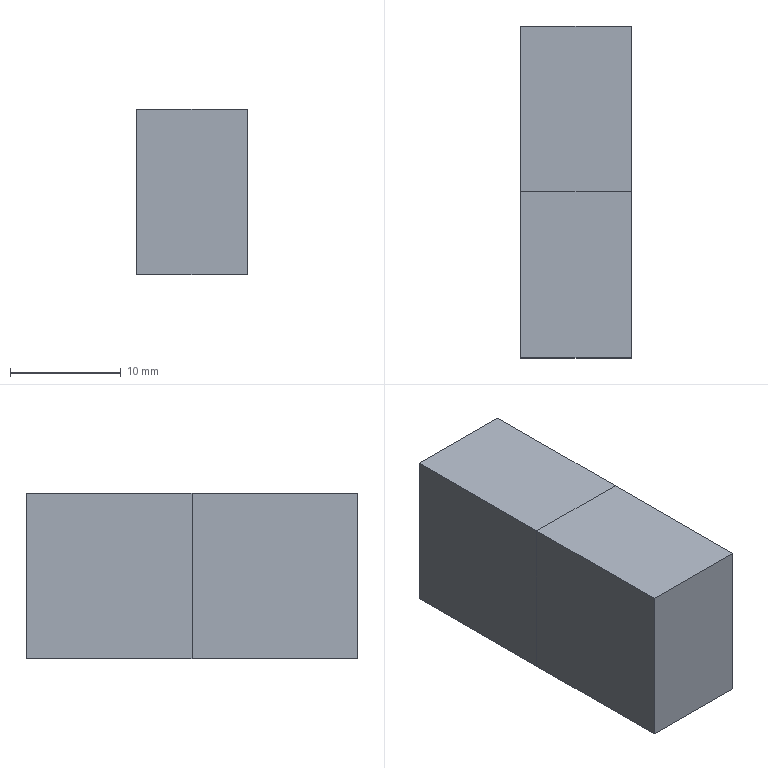Component | NX | 11_OBJECT_4 | 2 solids | 12 faces | box 10 x 30 x 15 mm | volume 4500 mm3 | plane 12
STEP:
#1=CARTESIAN_POINT('',(0.,0.,0.));
#2=DIRECTION('',(0.,0.,1.));
#3=DIRECTION('',(1.,0.,0.));
#4=AXIS2_PLACEMENT_3D('',#1,#2,#3);
#5=CARTESIAN_POINT('',(2050.,34.5,562.5));
#6=VERTEX_POINT('',#5);
#7=CARTESIAN_POINT('',(2050.,49.5,562.5));
#8=VERTEX_POINT('',#7);
#9=CARTESIAN_POINT('',(2050.,34.5,562.5));
#10=DIRECTION('',(0.,1.,0.));
#11=VECTOR('',#10,1.);
#12=LINE('',#9,#11);
#13=CARTESIAN_POINT('',(2060.,34.5,562.5));
#14=DIRECTION('',(0.,0.,1.));
#15=DIRECTION('',(0.,1.,0.));
#16=AXIS2_PLACEMENT_3D('',#13,#14,#15);
#17=PLANE('',#16);
#18=CARTESIAN_POINT('',(0.,10.));
#19=DIRECTION('',(1.,0.));
#20=VECTOR('',#19,1.);
#21=LINE('',#18,#20);
#22=(GEOMETRIC_REPRESENTATION_CONTEXT(2)PARAMETRIC_REPRESENTATION_CONTEXT()REPRESENTATION_CONTEXT('',''));
#23=DEFINITIONAL_REPRESENTATION('',(#21),#22);
#24=PCURVE('',#17,#23);
#25=CARTESIAN_POINT('',(2050.,34.5,562.5));
#26=DIRECTION('',(1.,0.,0.));
#27=DIRECTION('',(0.,1.,0.));
#28=AXIS2_PLACEMENT_3D('',#25,#26,#27);
#29=PLANE('',#28);
#30=CARTESIAN_POINT('',(0.,0.));
#31=DIRECTION('',(1.,0.));
#32=VECTOR('',#31,1.);
#33=LINE('',#30,#32);
#34=(GEOMETRIC_REPRESENTATION_CONTEXT(2)PARAMETRIC_REPRESENTATION_CONTEXT()REPRESENTATION_CONTEXT('',''));
#35=DEFINITIONAL_REPRESENTATION('',(#33),#34);
#36=PCURVE('',#29,#35);
#37=SURFACE_CURVE('',#12,(#24,#36),.PCURVE_S1.);
#38=EDGE_CURVE('',#6,#8,#37,.T.);
#39=ORIENTED_EDGE('',*,*,#38,.T.);
#40=CARTESIAN_POINT('',(2060.,49.5,562.5));
#41=VERTEX_POINT('',#40);
#42=CARTESIAN_POINT('',(2060.,49.5,562.5));
#43=DIRECTION('',(-1.,0.,0.));
#44=VECTOR('',#43,1.);
#45=LINE('',#42,#44);
#46=CARTESIAN_POINT('',(15.,0.));
#47=DIRECTION('',(0.,1.));
#48=VECTOR('',#47,1.);
#49=LINE('',#46,#48);
#50=(GEOMETRIC_REPRESENTATION_CONTEXT(2)PARAMETRIC_REPRESENTATION_CONTEXT()REPRESENTATION_CONTEXT('',''));
#51=DEFINITIONAL_REPRESENTATION('',(#49),#50);
#52=PCURVE('',#17,#51);
#53=CARTESIAN_POINT('',(2060.,49.5,562.5));
#54=DIRECTION('',(0.,-1.,0.));
#55=DIRECTION('',(0.,0.,1.));
#56=AXIS2_PLACEMENT_3D('',#53,#54,#55);
#57=PLANE('',#56);
#58=CARTESIAN_POINT('',(0.,0.));
#59=DIRECTION('',(0.,1.));
#60=VECTOR('',#59,1.);
#61=LINE('',#58,#60);
#62=(GEOMETRIC_REPRESENTATION_CONTEXT(2)PARAMETRIC_REPRESENTATION_CONTEXT()REPRESENTATION_CONTEXT('',''));
#63=DEFINITIONAL_REPRESENTATION('',(#61),#62);
#64=PCURVE('',#57,#63);
#65=SURFACE_CURVE('',#45,(#52,#64),.PCURVE_S1.);
#66=EDGE_CURVE('',#41,#8,#65,.T.);
#67=ORIENTED_EDGE('',*,*,#66,.F.);
#68=CARTESIAN_POINT('',(2060.,34.5,562.5));
#69=VERTEX_POINT('',#68);
#70=CARTESIAN_POINT('',(2060.,34.5,562.5));
#71=DIRECTION('',(0.,1.,0.));
#72=VECTOR('',#71,1.);
#73=LINE('',#70,#72);
#74=CARTESIAN_POINT('',(0.,0.));
#75=DIRECTION('',(1.,0.));
#76=VECTOR('',#75,1.);
#77=LINE('',#74,#76);
#78=(GEOMETRIC_REPRESENTATION_CONTEXT(2)PARAMETRIC_REPRESENTATION_CONTEXT()REPRESENTATION_CONTEXT('',''));
#79=DEFINITIONAL_REPRESENTATION('',(#77),#78);
#80=PCURVE('',#17,#79);
#81=CARTESIAN_POINT('',(2060.,34.5,562.5));
#82=DIRECTION('',(1.,0.,0.));
#83=DIRECTION('',(0.,1.,0.));
#84=AXIS2_PLACEMENT_3D('',#81,#82,#83);
#85=PLANE('',#84);
#86=CARTESIAN_POINT('',(0.,0.));
#87=DIRECTION('',(1.,0.));
#88=VECTOR('',#87,1.);
#89=LINE('',#86,#88);
#90=(GEOMETRIC_REPRESENTATION_CONTEXT(2)PARAMETRIC_REPRESENTATION_CONTEXT()REPRESENTATION_CONTEXT('',''));
#91=DEFINITIONAL_REPRESENTATION('',(#89),#90);
#92=PCURVE('',#85,#91);
#93=SURFACE_CURVE('',#73,(#80,#92),.PCURVE_S1.);
#94=EDGE_CURVE('',#69,#41,#93,.T.);
#95=ORIENTED_EDGE('',*,*,#94,.F.);
#96=CARTESIAN_POINT('',(2060.,34.5,562.5));
#97=DIRECTION('',(-1.,0.,0.));
#98=VECTOR('',#97,1.);
#99=LINE('',#96,#98);
#100=CARTESIAN_POINT('',(0.,0.));
#101=DIRECTION('',(0.,1.));
#102=VECTOR('',#101,1.);
#103=LINE('',#100,#102);
#104=(GEOMETRIC_REPRESENTATION_CONTEXT(2)PARAMETRIC_REPRESENTATION_CONTEXT()REPRESENTATION_CONTEXT('',''));
#105=DEFINITIONAL_REPRESENTATION('',(#103),#104);
#106=PCURVE('',#17,#105);
#107=CARTESIAN_POINT('',(2060.,34.5,577.5));
#108=DIRECTION('',(0.,1.,0.));
#109=DIRECTION('',(0.,0.,-1.));
#110=AXIS2_PLACEMENT_3D('',#107,#108,#109);
#111=PLANE('',#110);
#112=CARTESIAN_POINT('',(15.,0.));
#113=DIRECTION('',(0.,1.));
#114=VECTOR('',#113,1.);
#115=LINE('',#112,#114);
#116=(GEOMETRIC_REPRESENTATION_CONTEXT(2)PARAMETRIC_REPRESENTATION_CONTEXT()REPRESENTATION_CONTEXT('',''));
#117=DEFINITIONAL_REPRESENTATION('',(#115),#116);
#118=PCURVE('',#111,#117);
#119=SURFACE_CURVE('',#99,(#106,#118),.PCURVE_S1.);
#120=EDGE_CURVE('',#69,#6,#119,.T.);
#121=ORIENTED_EDGE('',*,*,#120,.T.);
#122=EDGE_LOOP('',(#39,#67,#95,#121));
#123=FACE_BOUND('',#122,.T.);
#124=ADVANCED_FACE('',(#123),#17,.F.);
#125=CARTESIAN_POINT('',(2050.,49.5,577.5));
#126=VERTEX_POINT('',#125);
#127=CARTESIAN_POINT('',(2050.,49.5,562.5));
#128=DIRECTION('',(0.,0.,1.));
#129=VECTOR('',#128,1.);
#130=LINE('',#127,#129);
#131=CARTESIAN_POINT('',(0.,10.));
#132=DIRECTION('',(1.,0.));
#133=VECTOR('',#132,1.);
#134=LINE('',#131,#133);
#135=(GEOMETRIC_REPRESENTATION_CONTEXT(2)PARAMETRIC_REPRESENTATION_CONTEXT()REPRESENTATION_CONTEXT('',''));
#136=DEFINITIONAL_REPRESENTATION('',(#134),#135);
#137=PCURVE('',#57,#136);
#138=CARTESIAN_POINT('',(15.,0.));
#139=DIRECTION('',(0.,1.));
#140=VECTOR('',#139,1.);
#141=LINE('',#138,#140);
#142=(GEOMETRIC_REPRESENTATION_CONTEXT(2)PARAMETRIC_REPRESENTATION_CONTEXT()REPRESENTATION_CONTEXT('',''));
#143=DEFINITIONAL_REPRESENTATION('',(#141),#142);
#144=PCURVE('',#29,#143);
#145=SURFACE_CURVE('',#130,(#137,#144),.PCURVE_S1.);
#146=EDGE_CURVE('',#8,#126,#145,.T.);
#147=ORIENTED_EDGE('',*,*,#146,.T.);
#148=CARTESIAN_POINT('',(2060.,49.5,577.5));
#149=VERTEX_POINT('',#148);
#150=CARTESIAN_POINT('',(2060.,49.5,577.5));
#151=DIRECTION('',(-1.,0.,0.));
#152=VECTOR('',#151,1.);
#153=LINE('',#150,#152);
#154=CARTESIAN_POINT('',(15.,0.));
#155=DIRECTION('',(0.,1.));
#156=VECTOR('',#155,1.);
#157=LINE('',#154,#156);
#158=(GEOMETRIC_REPRESENTATION_CONTEXT(2)PARAMETRIC_REPRESENTATION_CONTEXT()REPRESENTATION_CONTEXT('',''));
#159=DEFINITIONAL_REPRESENTATION('',(#157),#158);
#160=PCURVE('',#57,#159);
#161=CARTESIAN_POINT('',(2060.,49.5,577.5));
#162=DIRECTION('',(0.,0.,-1.));
#163=DIRECTION('',(0.,-1.,0.));
#164=AXIS2_PLACEMENT_3D('',#161,#162,#163);
#165=PLANE('',#164);
#166=CARTESIAN_POINT('',(0.,0.));
#167=DIRECTION('',(0.,1.));
#168=VECTOR('',#167,1.);
#169=LINE('',#166,#168);
#170=(GEOMETRIC_REPRESENTATION_CONTEXT(2)PARAMETRIC_REPRESENTATION_CONTEXT()REPRESENTATION_CONTEXT('',''));
#171=DEFINITIONAL_REPRESENTATION('',(#169),#170);
#172=PCURVE('',#165,#171);
#173=SURFACE_CURVE('',#153,(#160,#172),.PCURVE_S1.);
#174=EDGE_CURVE('',#149,#126,#173,.T.);
#175=ORIENTED_EDGE('',*,*,#174,.F.);
#176=CARTESIAN_POINT('',(2060.,49.5,562.5));
#177=DIRECTION('',(0.,0.,1.));
#178=VECTOR('',#177,1.);
#179=LINE('',#176,#178);
#180=CARTESIAN_POINT('',(0.,0.));
#181=DIRECTION('',(1.,0.));
#182=VECTOR('',#181,1.);
#183=LINE('',#180,#182);
#184=(GEOMETRIC_REPRESENTATION_CONTEXT(2)PARAMETRIC_REPRESENTATION_CONTEXT()REPRESENTATION_CONTEXT('',''));
#185=DEFINITIONAL_REPRESENTATION('',(#183),#184);
#186=PCURVE('',#57,#185);
#187=CARTESIAN_POINT('',(15.,0.));
#188=DIRECTION('',(0.,1.));
#189=VECTOR('',#188,1.);
#190=LINE('',#187,#189);
#191=(GEOMETRIC_REPRESENTATION_CONTEXT(2)PARAMETRIC_REPRESENTATION_CONTEXT()REPRESENTATION_CONTEXT('',''));
#192=DEFINITIONAL_REPRESENTATION('',(#190),#191);
#193=PCURVE('',#85,#192);
#194=SURFACE_CURVE('',#179,(#186,#193),.PCURVE_S1.);
#195=EDGE_CURVE('',#41,#149,#194,.T.);
#196=ORIENTED_EDGE('',*,*,#195,.F.);
#197=ORIENTED_EDGE('',*,*,#66,.T.);
#198=EDGE_LOOP('',(#147,#175,#196,#197));
#199=FACE_BOUND('',#198,.T.);
#200=ADVANCED_FACE('',(#199),#57,.F.);
#201=CARTESIAN_POINT('',(2050.,34.5,577.5));
#202=VERTEX_POINT('',#201);
#203=CARTESIAN_POINT('',(2050.,49.5,577.5));
#204=DIRECTION('',(0.,-1.,0.));
#205=VECTOR('',#204,1.);
#206=LINE('',#203,#205);
#207=CARTESIAN_POINT('',(0.,10.));
#208=DIRECTION('',(1.,0.));
#209=VECTOR('',#208,1.);
#210=LINE('',#207,#209);
#211=(GEOMETRIC_REPRESENTATION_CONTEXT(2)PARAMETRIC_REPRESENTATION_CONTEXT()REPRESENTATION_CONTEXT('',''));
#212=DEFINITIONAL_REPRESENTATION('',(#210),#211);
#213=PCURVE('',#165,#212);
#214=CARTESIAN_POINT('',(15.,15.));
#215=DIRECTION('',(-1.,0.));
#216=VECTOR('',#215,1.);
#217=LINE('',#214,#216);
#218=(GEOMETRIC_REPRESENTATION_CONTEXT(2)PARAMETRIC_REPRESENTATION_CONTEXT()REPRESENTATION_CONTEXT('',''));
#219=DEFINITIONAL_REPRESENTATION('',(#217),#218);
#220=PCURVE('',#29,#219);
#221=SURFACE_CURVE('',#206,(#213,#220),.PCURVE_S1.);
#222=EDGE_CURVE('',#126,#202,#221,.T.);
#223=ORIENTED_EDGE('',*,*,#222,.T.);
#224=CARTESIAN_POINT('',(2060.,34.5,577.5));
#225=VERTEX_POINT('',#224);
#226=CARTESIAN_POINT('',(2060.,34.5,577.5));
#227=DIRECTION('',(-1.,0.,0.));
#228=VECTOR('',#227,1.);
#229=LINE('',#226,#228);
#230=CARTESIAN_POINT('',(15.,0.));
#231=DIRECTION('',(0.,1.));
#232=VECTOR('',#231,1.);
#233=LINE('',#230,#232);
#234=(GEOMETRIC_REPRESENTATION_CONTEXT(2)PARAMETRIC_REPRESENTATION_CONTEXT()REPRESENTATION_CONTEXT('',''));
#235=DEFINITIONAL_REPRESENTATION('',(#233),#234);
#236=PCURVE('',#165,#235);
#237=CARTESIAN_POINT('',(0.,0.));
#238=DIRECTION('',(0.,1.));
#239=VECTOR('',#238,1.);
#240=LINE('',#237,#239);
#241=(GEOMETRIC_REPRESENTATION_CONTEXT(2)PARAMETRIC_REPRESENTATION_CONTEXT()REPRESENTATION_CONTEXT('',''));
#242=DEFINITIONAL_REPRESENTATION('',(#240),#241);
#243=PCURVE('',#111,#242);
#244=SURFACE_CURVE('',#229,(#236,#243),.PCURVE_S1.);
#245=EDGE_CURVE('',#225,#202,#244,.T.);
#246=ORIENTED_EDGE('',*,*,#245,.F.);
#247=CARTESIAN_POINT('',(2060.,49.5,577.5));
#248=DIRECTION('',(0.,-1.,0.));
#249=VECTOR('',#248,1.);
#250=LINE('',#247,#249);
#251=CARTESIAN_POINT('',(0.,0.));
#252=DIRECTION('',(1.,0.));
#253=VECTOR('',#252,1.);
#254=LINE('',#251,#253);
#255=(GEOMETRIC_REPRESENTATION_CONTEXT(2)PARAMETRIC_REPRESENTATION_CONTEXT()REPRESENTATION_CONTEXT('',''));
#256=DEFINITIONAL_REPRESENTATION('',(#254),#255);
#257=PCURVE('',#165,#256);
#258=CARTESIAN_POINT('',(15.,15.));
#259=DIRECTION('',(-1.,0.));
#260=VECTOR('',#259,1.);
#261=LINE('',#258,#260);
#262=(GEOMETRIC_REPRESENTATION_CONTEXT(2)PARAMETRIC_REPRESENTATION_CONTEXT()REPRESENTATION_CONTEXT('',''));
#263=DEFINITIONAL_REPRESENTATION('',(#261),#262);
#264=PCURVE('',#85,#263);
#265=SURFACE_CURVE('',#250,(#257,#264),.PCURVE_S1.);
#266=EDGE_CURVE('',#149,#225,#265,.T.);
#267=ORIENTED_EDGE('',*,*,#266,.F.);
#268=ORIENTED_EDGE('',*,*,#174,.T.);
#269=EDGE_LOOP('',(#223,#246,#267,#268));
#270=FACE_BOUND('',#269,.T.);
#271=ADVANCED_FACE('',(#270),#165,.F.);
#272=CARTESIAN_POINT('',(2050.,34.5,577.5));
#273=DIRECTION('',(0.,0.,-1.));
#274=VECTOR('',#273,1.);
#275=LINE('',#272,#274);
#276=CARTESIAN_POINT('',(0.,10.));
#277=DIRECTION('',(1.,0.));
#278=VECTOR('',#277,1.);
#279=LINE('',#276,#278);
#280=(GEOMETRIC_REPRESENTATION_CONTEXT(2)PARAMETRIC_REPRESENTATION_CONTEXT()REPRESENTATION_CONTEXT('',''));
#281=DEFINITIONAL_REPRESENTATION('',(#279),#280);
#282=PCURVE('',#111,#281);
#283=CARTESIAN_POINT('',(0.,15.));
#284=DIRECTION('',(0.,-1.));
#285=VECTOR('',#284,1.);
#286=LINE('',#283,#285);
#287=(GEOMETRIC_REPRESENTATION_CONTEXT(2)PARAMETRIC_REPRESENTATION_CONTEXT()REPRESENTATION_CONTEXT('',''));
#288=DEFINITIONAL_REPRESENTATION('',(#286),#287);
#289=PCURVE('',#29,#288);
#290=SURFACE_CURVE('',#275,(#282,#289),.PCURVE_S1.);
#291=EDGE_CURVE('',#202,#6,#290,.T.);
#292=ORIENTED_EDGE('',*,*,#291,.T.);
#293=ORIENTED_EDGE('',*,*,#120,.F.);
#294=CARTESIAN_POINT('',(2060.,34.5,577.5));
#295=DIRECTION('',(0.,0.,-1.));
#296=VECTOR('',#295,1.);
#297=LINE('',#294,#296);
#298=CARTESIAN_POINT('',(0.,0.));
#299=DIRECTION('',(1.,0.));
#300=VECTOR('',#299,1.);
#301=LINE('',#298,#300);
#302=(GEOMETRIC_REPRESENTATION_CONTEXT(2)PARAMETRIC_REPRESENTATION_CONTEXT()REPRESENTATION_CONTEXT('',''));
#303=DEFINITIONAL_REPRESENTATION('',(#301),#302);
#304=PCURVE('',#111,#303);
#305=CARTESIAN_POINT('',(0.,15.));
#306=DIRECTION('',(0.,-1.));
#307=VECTOR('',#306,1.);
#308=LINE('',#305,#307);
#309=(GEOMETRIC_REPRESENTATION_CONTEXT(2)PARAMETRIC_REPRESENTATION_CONTEXT()REPRESENTATION_CONTEXT('',''));
#310=DEFINITIONAL_REPRESENTATION('',(#308),#309);
#311=PCURVE('',#85,#310);
#312=SURFACE_CURVE('',#297,(#304,#311),.PCURVE_S1.);
#313=EDGE_CURVE('',#225,#69,#312,.T.);
#314=ORIENTED_EDGE('',*,*,#313,.F.);
#315=ORIENTED_EDGE('',*,*,#245,.T.);
#316=EDGE_LOOP('',(#292,#293,#314,#315));
#317=FACE_BOUND('',#316,.T.);
#318=ADVANCED_FACE('',(#317),#111,.F.);
#319=ORIENTED_EDGE('',*,*,#94,.T.);
#320=ORIENTED_EDGE('',*,*,#195,.T.);
#321=ORIENTED_EDGE('',*,*,#266,.T.);
#322=ORIENTED_EDGE('',*,*,#313,.T.);
#323=EDGE_LOOP('',(#319,#320,#321,#322));
#324=FACE_BOUND('',#323,.T.);
#325=ADVANCED_FACE('',(#324),#85,.T.);
#326=ORIENTED_EDGE('',*,*,#38,.F.);
#327=ORIENTED_EDGE('',*,*,#291,.F.);
#328=ORIENTED_EDGE('',*,*,#222,.F.);
#329=ORIENTED_EDGE('',*,*,#146,.F.);
#330=EDGE_LOOP('',(#326,#327,#328,#329));
#331=FACE_BOUND('',#330,.T.);
#332=ADVANCED_FACE('',(#331),#29,.F.);
#333=CLOSED_SHELL('',(#124,#200,#271,#318,#325,#332));
#334=MANIFOLD_SOLID_BREP('',#333);
#335=(LENGTH_UNIT()NAMED_UNIT(*)SI_UNIT(.MILLI.,.METRE.));
#336=UNCERTAINTY_MEASURE_WITH_UNIT(LENGTH_MEASURE(0.0000001),#335,'','');
#337=(NAMED_UNIT(*)PLANE_ANGLE_UNIT()SI_UNIT($,.RADIAN.));
#338=(NAMED_UNIT(*)SI_UNIT($,.STERADIAN.)SOLID_ANGLE_UNIT());
#339=(GEOMETRIC_REPRESENTATION_CONTEXT(3)GLOBAL_UNCERTAINTY_ASSIGNED_CONTEXT((#336))GLOBAL_UNIT_ASSIGNED_CONTEXT((#335,#337,#338))REPRESENTATION_CONTEXT('',''));
#340=ADVANCED_BREP_SHAPE_REPRESENTATION('',(#4,#334),#339);
#341=CARTESIAN_POINT('',(0.,0.,0.));
#342=DIRECTION('',(0.,0.,1.));
#343=DIRECTION('',(1.,0.,0.));
#344=AXIS2_PLACEMENT_3D('',#341,#342,#343);
#345=CARTESIAN_POINT('',(0.,0.,0.));
#346=DIRECTION('',(0.,0.,1.));
#347=DIRECTION('',(1.,0.,0.));
#348=AXIS2_PLACEMENT_3D('',#345,#346,#347);
#349=(LENGTH_UNIT()NAMED_UNIT(*)SI_UNIT(.MILLI.,.METRE.));
#350=UNCERTAINTY_MEASURE_WITH_UNIT(LENGTH_MEASURE(0.0000001),#349,'','');
#351=(NAMED_UNIT(*)PLANE_ANGLE_UNIT()SI_UNIT($,.RADIAN.));
#352=(NAMED_UNIT(*)SI_UNIT($,.STERADIAN.)SOLID_ANGLE_UNIT());
#353=(GEOMETRIC_REPRESENTATION_CONTEXT(3)GLOBAL_UNCERTAINTY_ASSIGNED_CONTEXT((#350))GLOBAL_UNIT_ASSIGNED_CONTEXT((#349,#351,#352))REPRESENTATION_CONTEXT('',''));
#354=SHAPE_REPRESENTATION('',(#4,#344,#348),#353);
#355=ITEM_DEFINED_TRANSFORMATION('','',#4,#344);
#356=(REPRESENTATION_RELATIONSHIP('','',#340,#354)REPRESENTATION_RELATIONSHIP_WITH_TRANSFORMATION(#355)SHAPE_REPRESENTATION_RELATIONSHIP());
#357=CARTESIAN_POINT('',(2050.,19.5,562.5));
#358=VERTEX_POINT('',#357);
#359=CARTESIAN_POINT('',(2050.,34.5,562.5));
#360=VERTEX_POINT('',#359);
#361=CARTESIAN_POINT('',(2050.,19.5,562.5));
#362=DIRECTION('',(0.,1.,0.));
#363=VECTOR('',#362,1.);
#364=LINE('',#361,#363);
#365=CARTESIAN_POINT('',(2060.,19.5,562.5));
#366=DIRECTION('',(0.,0.,1.));
#367=DIRECTION('',(0.,1.,0.));
#368=AXIS2_PLACEMENT_3D('',#365,#366,#367);
#369=PLANE('',#368);
#370=CARTESIAN_POINT('',(0.,10.));
#371=DIRECTION('',(1.,0.));
#372=VECTOR('',#371,1.);
#373=LINE('',#370,#372);
#374=(GEOMETRIC_REPRESENTATION_CONTEXT(2)PARAMETRIC_REPRESENTATION_CONTEXT()REPRESENTATION_CONTEXT('',''));
#375=DEFINITIONAL_REPRESENTATION('',(#373),#374);
#376=PCURVE('',#369,#375);
#377=CARTESIAN_POINT('',(2050.,19.5,562.5));
#378=DIRECTION('',(1.,0.,0.));
#379=DIRECTION('',(0.,1.,0.));
#380=AXIS2_PLACEMENT_3D('',#377,#378,#379);
#381=PLANE('',#380);
#382=CARTESIAN_POINT('',(0.,0.));
#383=DIRECTION('',(1.,0.));
#384=VECTOR('',#383,1.);
#385=LINE('',#382,#384);
#386=(GEOMETRIC_REPRESENTATION_CONTEXT(2)PARAMETRIC_REPRESENTATION_CONTEXT()REPRESENTATION_CONTEXT('',''));
#387=DEFINITIONAL_REPRESENTATION('',(#385),#386);
#388=PCURVE('',#381,#387);
#389=SURFACE_CURVE('',#364,(#376,#388),.PCURVE_S1.);
#390=EDGE_CURVE('',#358,#360,#389,.T.);
#391=ORIENTED_EDGE('',*,*,#390,.T.);
#392=CARTESIAN_POINT('',(2060.,34.5,562.5));
#393=VERTEX_POINT('',#392);
#394=CARTESIAN_POINT('',(2060.,34.5,562.5));
#395=DIRECTION('',(-1.,0.,0.));
#396=VECTOR('',#395,1.);
#397=LINE('',#394,#396);
#398=CARTESIAN_POINT('',(15.,0.));
#399=DIRECTION('',(0.,1.));
#400=VECTOR('',#399,1.);
#401=LINE('',#398,#400);
#402=(GEOMETRIC_REPRESENTATION_CONTEXT(2)PARAMETRIC_REPRESENTATION_CONTEXT()REPRESENTATION_CONTEXT('',''));
#403=DEFINITIONAL_REPRESENTATION('',(#401),#402);
#404=PCURVE('',#369,#403);
#405=CARTESIAN_POINT('',(2060.,34.5,562.5));
#406=DIRECTION('',(0.,-1.,0.));
#407=DIRECTION('',(0.,0.,1.));
#408=AXIS2_PLACEMENT_3D('',#405,#406,#407);
#409=PLANE('',#408);
#410=CARTESIAN_POINT('',(0.,0.));
#411=DIRECTION('',(0.,1.));
#412=VECTOR('',#411,1.);
#413=LINE('',#410,#412);
#414=(GEOMETRIC_REPRESENTATION_CONTEXT(2)PARAMETRIC_REPRESENTATION_CONTEXT()REPRESENTATION_CONTEXT('',''));
#415=DEFINITIONAL_REPRESENTATION('',(#413),#414);
#416=PCURVE('',#409,#415);
#417=SURFACE_CURVE('',#397,(#404,#416),.PCURVE_S1.);
#418=EDGE_CURVE('',#393,#360,#417,.T.);
#419=ORIENTED_EDGE('',*,*,#418,.F.);
#420=CARTESIAN_POINT('',(2060.,19.5,562.5));
#421=VERTEX_POINT('',#420);
#422=CARTESIAN_POINT('',(2060.,19.5,562.5));
#423=DIRECTION('',(0.,1.,0.));
#424=VECTOR('',#423,1.);
#425=LINE('',#422,#424);
#426=CARTESIAN_POINT('',(0.,0.));
#427=DIRECTION('',(1.,0.));
#428=VECTOR('',#427,1.);
#429=LINE('',#426,#428);
#430=(GEOMETRIC_REPRESENTATION_CONTEXT(2)PARAMETRIC_REPRESENTATION_CONTEXT()REPRESENTATION_CONTEXT('',''));
#431=DEFINITIONAL_REPRESENTATION('',(#429),#430);
#432=PCURVE('',#369,#431);
#433=CARTESIAN_POINT('',(2060.,19.5,562.5));
#434=DIRECTION('',(1.,0.,0.));
#435=DIRECTION('',(0.,1.,0.));
#436=AXIS2_PLACEMENT_3D('',#433,#434,#435);
#437=PLANE('',#436);
#438=CARTESIAN_POINT('',(0.,0.));
#439=DIRECTION('',(1.,0.));
#440=VECTOR('',#439,1.);
#441=LINE('',#438,#440);
#442=(GEOMETRIC_REPRESENTATION_CONTEXT(2)PARAMETRIC_REPRESENTATION_CONTEXT()REPRESENTATION_CONTEXT('',''));
#443=DEFINITIONAL_REPRESENTATION('',(#441),#442);
#444=PCURVE('',#437,#443);
#445=SURFACE_CURVE('',#425,(#432,#444),.PCURVE_S1.);
#446=EDGE_CURVE('',#421,#393,#445,.T.);
#447=ORIENTED_EDGE('',*,*,#446,.F.);
#448=CARTESIAN_POINT('',(2060.,19.5,562.5));
#449=DIRECTION('',(-1.,0.,0.));
#450=VECTOR('',#449,1.);
#451=LINE('',#448,#450);
#452=CARTESIAN_POINT('',(0.,0.));
#453=DIRECTION('',(0.,1.));
#454=VECTOR('',#453,1.);
#455=LINE('',#452,#454);
#456=(GEOMETRIC_REPRESENTATION_CONTEXT(2)PARAMETRIC_REPRESENTATION_CONTEXT()REPRESENTATION_CONTEXT('',''));
#457=DEFINITIONAL_REPRESENTATION('',(#455),#456);
#458=PCURVE('',#369,#457);
#459=CARTESIAN_POINT('',(2060.,19.5,577.5));
#460=DIRECTION('',(0.,1.,0.));
#461=DIRECTION('',(0.,0.,-1.));
#462=AXIS2_PLACEMENT_3D('',#459,#460,#461);
#463=PLANE('',#462);
#464=CARTESIAN_POINT('',(15.,0.));
#465=DIRECTION('',(0.,1.));
#466=VECTOR('',#465,1.);
#467=LINE('',#464,#466);
#468=(GEOMETRIC_REPRESENTATION_CONTEXT(2)PARAMETRIC_REPRESENTATION_CONTEXT()REPRESENTATION_CONTEXT('',''));
#469=DEFINITIONAL_REPRESENTATION('',(#467),#468);
#470=PCURVE('',#463,#469);
#471=SURFACE_CURVE('',#451,(#458,#470),.PCURVE_S1.);
#472=EDGE_CURVE('',#421,#358,#471,.T.);
#473=ORIENTED_EDGE('',*,*,#472,.T.);
#474=EDGE_LOOP('',(#391,#419,#447,#473));
#475=FACE_BOUND('',#474,.T.);
#476=ADVANCED_FACE('',(#475),#369,.F.);
#477=CARTESIAN_POINT('',(2050.,34.5,577.5));
#478=VERTEX_POINT('',#477);
#479=CARTESIAN_POINT('',(2050.,34.5,562.5));
#480=DIRECTION('',(0.,0.,1.));
#481=VECTOR('',#480,1.);
#482=LINE('',#479,#481);
#483=CARTESIAN_POINT('',(0.,10.));
#484=DIRECTION('',(1.,0.));
#485=VECTOR('',#484,1.);
#486=LINE('',#483,#485);
#487=(GEOMETRIC_REPRESENTATION_CONTEXT(2)PARAMETRIC_REPRESENTATION_CONTEXT()REPRESENTATION_CONTEXT('',''));
#488=DEFINITIONAL_REPRESENTATION('',(#486),#487);
#489=PCURVE('',#409,#488);
#490=CARTESIAN_POINT('',(15.,0.));
#491=DIRECTION('',(0.,1.));
#492=VECTOR('',#491,1.);
#493=LINE('',#490,#492);
#494=(GEOMETRIC_REPRESENTATION_CONTEXT(2)PARAMETRIC_REPRESENTATION_CONTEXT()REPRESENTATION_CONTEXT('',''));
#495=DEFINITIONAL_REPRESENTATION('',(#493),#494);
#496=PCURVE('',#381,#495);
#497=SURFACE_CURVE('',#482,(#489,#496),.PCURVE_S1.);
#498=EDGE_CURVE('',#360,#478,#497,.T.);
#499=ORIENTED_EDGE('',*,*,#498,.T.);
#500=CARTESIAN_POINT('',(2060.,34.5,577.5));
#501=VERTEX_POINT('',#500);
#502=CARTESIAN_POINT('',(2060.,34.5,577.5));
#503=DIRECTION('',(-1.,0.,0.));
#504=VECTOR('',#503,1.);
#505=LINE('',#502,#504);
#506=CARTESIAN_POINT('',(15.,0.));
#507=DIRECTION('',(0.,1.));
#508=VECTOR('',#507,1.);
#509=LINE('',#506,#508);
#510=(GEOMETRIC_REPRESENTATION_CONTEXT(2)PARAMETRIC_REPRESENTATION_CONTEXT()REPRESENTATION_CONTEXT('',''));
#511=DEFINITIONAL_REPRESENTATION('',(#509),#510);
#512=PCURVE('',#409,#511);
#513=CARTESIAN_POINT('',(2060.,34.5,577.5));
#514=DIRECTION('',(0.,0.,-1.));
#515=DIRECTION('',(0.,-1.,0.));
#516=AXIS2_PLACEMENT_3D('',#513,#514,#515);
#517=PLANE('',#516);
#518=CARTESIAN_POINT('',(0.,0.));
#519=DIRECTION('',(0.,1.));
#520=VECTOR('',#519,1.);
#521=LINE('',#518,#520);
#522=(GEOMETRIC_REPRESENTATION_CONTEXT(2)PARAMETRIC_REPRESENTATION_CONTEXT()REPRESENTATION_CONTEXT('',''));
#523=DEFINITIONAL_REPRESENTATION('',(#521),#522);
#524=PCURVE('',#517,#523);
#525=SURFACE_CURVE('',#505,(#512,#524),.PCURVE_S1.);
#526=EDGE_CURVE('',#501,#478,#525,.T.);
#527=ORIENTED_EDGE('',*,*,#526,.F.);
#528=CARTESIAN_POINT('',(2060.,34.5,562.5));
#529=DIRECTION('',(0.,0.,1.));
#530=VECTOR('',#529,1.);
#531=LINE('',#528,#530);
#532=CARTESIAN_POINT('',(0.,0.));
#533=DIRECTION('',(1.,0.));
#534=VECTOR('',#533,1.);
#535=LINE('',#532,#534);
#536=(GEOMETRIC_REPRESENTATION_CONTEXT(2)PARAMETRIC_REPRESENTATION_CONTEXT()REPRESENTATION_CONTEXT('',''));
#537=DEFINITIONAL_REPRESENTATION('',(#535),#536);
#538=PCURVE('',#409,#537);
#539=CARTESIAN_POINT('',(15.,0.));
#540=DIRECTION('',(0.,1.));
#541=VECTOR('',#540,1.);
#542=LINE('',#539,#541);
#543=(GEOMETRIC_REPRESENTATION_CONTEXT(2)PARAMETRIC_REPRESENTATION_CONTEXT()REPRESENTATION_CONTEXT('',''));
#544=DEFINITIONAL_REPRESENTATION('',(#542),#543);
#545=PCURVE('',#437,#544);
#546=SURFACE_CURVE('',#531,(#538,#545),.PCURVE_S1.);
#547=EDGE_CURVE('',#393,#501,#546,.T.);
#548=ORIENTED_EDGE('',*,*,#547,.F.);
#549=ORIENTED_EDGE('',*,*,#418,.T.);
#550=EDGE_LOOP('',(#499,#527,#548,#549));
#551=FACE_BOUND('',#550,.T.);
#552=ADVANCED_FACE('',(#551),#409,.F.);
#553=CARTESIAN_POINT('',(2050.,19.5,577.5));
#554=VERTEX_POINT('',#553);
#555=CARTESIAN_POINT('',(2050.,34.5,577.5));
#556=DIRECTION('',(0.,-1.,0.));
#557=VECTOR('',#556,1.);
#558=LINE('',#555,#557);
#559=CARTESIAN_POINT('',(0.,10.));
#560=DIRECTION('',(1.,0.));
#561=VECTOR('',#560,1.);
#562=LINE('',#559,#561);
#563=(GEOMETRIC_REPRESENTATION_CONTEXT(2)PARAMETRIC_REPRESENTATION_CONTEXT()REPRESENTATION_CONTEXT('',''));
#564=DEFINITIONAL_REPRESENTATION('',(#562),#563);
#565=PCURVE('',#517,#564);
#566=CARTESIAN_POINT('',(15.,15.));
#567=DIRECTION('',(-1.,0.));
#568=VECTOR('',#567,1.);
#569=LINE('',#566,#568);
#570=(GEOMETRIC_REPRESENTATION_CONTEXT(2)PARAMETRIC_REPRESENTATION_CONTEXT()REPRESENTATION_CONTEXT('',''));
#571=DEFINITIONAL_REPRESENTATION('',(#569),#570);
#572=PCURVE('',#381,#571);
#573=SURFACE_CURVE('',#558,(#565,#572),.PCURVE_S1.);
#574=EDGE_CURVE('',#478,#554,#573,.T.);
#575=ORIENTED_EDGE('',*,*,#574,.T.);
#576=CARTESIAN_POINT('',(2060.,19.5,577.5));
#577=VERTEX_POINT('',#576);
#578=CARTESIAN_POINT('',(2060.,19.5,577.5));
#579=DIRECTION('',(-1.,0.,0.));
#580=VECTOR('',#579,1.);
#581=LINE('',#578,#580);
#582=CARTESIAN_POINT('',(15.,0.));
#583=DIRECTION('',(0.,1.));
#584=VECTOR('',#583,1.);
#585=LINE('',#582,#584);
#586=(GEOMETRIC_REPRESENTATION_CONTEXT(2)PARAMETRIC_REPRESENTATION_CONTEXT()REPRESENTATION_CONTEXT('',''));
#587=DEFINITIONAL_REPRESENTATION('',(#585),#586);
#588=PCURVE('',#517,#587);
#589=CARTESIAN_POINT('',(0.,0.));
#590=DIRECTION('',(0.,1.));
#591=VECTOR('',#590,1.);
#592=LINE('',#589,#591);
#593=(GEOMETRIC_REPRESENTATION_CONTEXT(2)PARAMETRIC_REPRESENTATION_CONTEXT()REPRESENTATION_CONTEXT('',''));
#594=DEFINITIONAL_REPRESENTATION('',(#592),#593);
#595=PCURVE('',#463,#594);
#596=SURFACE_CURVE('',#581,(#588,#595),.PCURVE_S1.);
#597=EDGE_CURVE('',#577,#554,#596,.T.);
#598=ORIENTED_EDGE('',*,*,#597,.F.);
#599=CARTESIAN_POINT('',(2060.,34.5,577.5));
#600=DIRECTION('',(0.,-1.,0.));
#601=VECTOR('',#600,1.);
#602=LINE('',#599,#601);
#603=CARTESIAN_POINT('',(0.,0.));
#604=DIRECTION('',(1.,0.));
#605=VECTOR('',#604,1.);
#606=LINE('',#603,#605);
#607=(GEOMETRIC_REPRESENTATION_CONTEXT(2)PARAMETRIC_REPRESENTATION_CONTEXT()REPRESENTATION_CONTEXT('',''));
#608=DEFINITIONAL_REPRESENTATION('',(#606),#607);
#609=PCURVE('',#517,#608);
#610=CARTESIAN_POINT('',(15.,15.));
#611=DIRECTION('',(-1.,0.));
#612=VECTOR('',#611,1.);
#613=LINE('',#610,#612);
#614=(GEOMETRIC_REPRESENTATION_CONTEXT(2)PARAMETRIC_REPRESENTATION_CONTEXT()REPRESENTATION_CONTEXT('',''));
#615=DEFINITIONAL_REPRESENTATION('',(#613),#614);
#616=PCURVE('',#437,#615);
#617=SURFACE_CURVE('',#602,(#609,#616),.PCURVE_S1.);
#618=EDGE_CURVE('',#501,#577,#617,.T.);
#619=ORIENTED_EDGE('',*,*,#618,.F.);
#620=ORIENTED_EDGE('',*,*,#526,.T.);
#621=EDGE_LOOP('',(#575,#598,#619,#620));
#622=FACE_BOUND('',#621,.T.);
#623=ADVANCED_FACE('',(#622),#517,.F.);
#624=CARTESIAN_POINT('',(2050.,19.5,577.5));
#625=DIRECTION('',(0.,0.,-1.));
#626=VECTOR('',#625,1.);
#627=LINE('',#624,#626);
#628=CARTESIAN_POINT('',(0.,10.));
#629=DIRECTION('',(1.,0.));
#630=VECTOR('',#629,1.);
#631=LINE('',#628,#630);
#632=(GEOMETRIC_REPRESENTATION_CONTEXT(2)PARAMETRIC_REPRESENTATION_CONTEXT()REPRESENTATION_CONTEXT('',''));
#633=DEFINITIONAL_REPRESENTATION('',(#631),#632);
#634=PCURVE('',#463,#633);
#635=CARTESIAN_POINT('',(0.,15.));
#636=DIRECTION('',(0.,-1.));
#637=VECTOR('',#636,1.);
#638=LINE('',#635,#637);
#639=(GEOMETRIC_REPRESENTATION_CONTEXT(2)PARAMETRIC_REPRESENTATION_CONTEXT()REPRESENTATION_CONTEXT('',''));
#640=DEFINITIONAL_REPRESENTATION('',(#638),#639);
#641=PCURVE('',#381,#640);
#642=SURFACE_CURVE('',#627,(#634,#641),.PCURVE_S1.);
#643=EDGE_CURVE('',#554,#358,#642,.T.);
#644=ORIENTED_EDGE('',*,*,#643,.T.);
#645=ORIENTED_EDGE('',*,*,#472,.F.);
#646=CARTESIAN_POINT('',(2060.,19.5,577.5));
#647=DIRECTION('',(0.,0.,-1.));
#648=VECTOR('',#647,1.);
#649=LINE('',#646,#648);
#650=CARTESIAN_POINT('',(0.,0.));
#651=DIRECTION('',(1.,0.));
#652=VECTOR('',#651,1.);
#653=LINE('',#650,#652);
#654=(GEOMETRIC_REPRESENTATION_CONTEXT(2)PARAMETRIC_REPRESENTATION_CONTEXT()REPRESENTATION_CONTEXT('',''));
#655=DEFINITIONAL_REPRESENTATION('',(#653),#654);
#656=PCURVE('',#463,#655);
#657=CARTESIAN_POINT('',(0.,15.));
#658=DIRECTION('',(0.,-1.));
#659=VECTOR('',#658,1.);
#660=LINE('',#657,#659);
#661=(GEOMETRIC_REPRESENTATION_CONTEXT(2)PARAMETRIC_REPRESENTATION_CONTEXT()REPRESENTATION_CONTEXT('',''));
#662=DEFINITIONAL_REPRESENTATION('',(#660),#661);
#663=PCURVE('',#437,#662);
#664=SURFACE_CURVE('',#649,(#656,#663),.PCURVE_S1.);
#665=EDGE_CURVE('',#577,#421,#664,.T.);
#666=ORIENTED_EDGE('',*,*,#665,.F.);
#667=ORIENTED_EDGE('',*,*,#597,.T.);
#668=EDGE_LOOP('',(#644,#645,#666,#667));
#669=FACE_BOUND('',#668,.T.);
#670=ADVANCED_FACE('',(#669),#463,.F.);
#671=ORIENTED_EDGE('',*,*,#446,.T.);
#672=ORIENTED_EDGE('',*,*,#547,.T.);
#673=ORIENTED_EDGE('',*,*,#618,.T.);
#674=ORIENTED_EDGE('',*,*,#665,.T.);
#675=EDGE_LOOP('',(#671,#672,#673,#674));
#676=FACE_BOUND('',#675,.T.);
#677=ADVANCED_FACE('',(#676),#437,.T.);
#678=ORIENTED_EDGE('',*,*,#390,.F.);
#679=ORIENTED_EDGE('',*,*,#643,.F.);
#680=ORIENTED_EDGE('',*,*,#574,.F.);
#681=ORIENTED_EDGE('',*,*,#498,.F.);
#682=EDGE_LOOP('',(#678,#679,#680,#681));
#683=FACE_BOUND('',#682,.T.);
#684=ADVANCED_FACE('',(#683),#381,.F.);
#685=CLOSED_SHELL('',(#476,#552,#623,#670,#677,#684));
#686=MANIFOLD_SOLID_BREP('',#685);
#687=(LENGTH_UNIT()NAMED_UNIT(*)SI_UNIT(.MILLI.,.METRE.));
#688=UNCERTAINTY_MEASURE_WITH_UNIT(LENGTH_MEASURE(0.0000001),#687,'','');
#689=(NAMED_UNIT(*)PLANE_ANGLE_UNIT()SI_UNIT($,.RADIAN.));
#690=(NAMED_UNIT(*)SI_UNIT($,.STERADIAN.)SOLID_ANGLE_UNIT());
#691=(GEOMETRIC_REPRESENTATION_CONTEXT(3)GLOBAL_UNCERTAINTY_ASSIGNED_CONTEXT((#688))GLOBAL_UNIT_ASSIGNED_CONTEXT((#687,#689,#690))REPRESENTATION_CONTEXT('',''));
#692=ADVANCED_BREP_SHAPE_REPRESENTATION('',(#4,#686),#691);
#693=ITEM_DEFINED_TRANSFORMATION('','',#4,#348);
#694=(REPRESENTATION_RELATIONSHIP('','',#692,#354)REPRESENTATION_RELATIONSHIP_WITH_TRANSFORMATION(#693)SHAPE_REPRESENTATION_RELATIONSHIP());